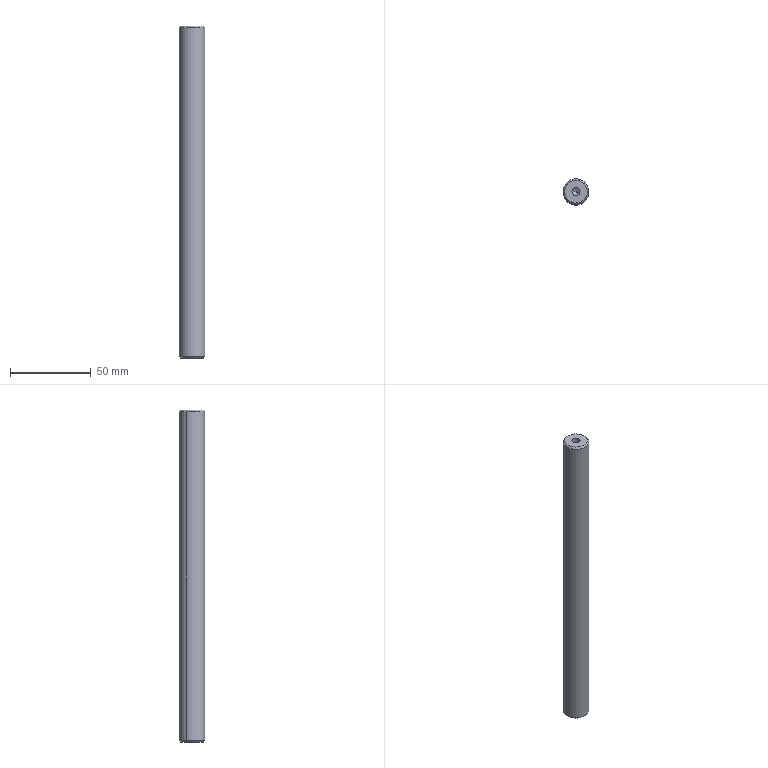Component | SolidWorks | DZ.KX.203-TC1505-30-09-01-05-02-1 | 1 solid | 16 faces | box 16 x 16 x 205 mm | volume 40443 mm3 | cone 8 | cylinder 6 | plane 2 | commonest cylinder face diameters 5 x4 16 x2 | material Malleable Cast Iron
build123d program:
from build123d import *

# Parameters (mm, degrees)
SKETCH1_R             = 8
BOSS_EXTRUDE1_DEPTH   = 205
M6_TAPPED_HOLE1_D     = 5
M6_TAPPED_HOLE1_DEPTH = 18
M6_TAPPED_HOLE1_TIP   = 1.502
M6_TAPPED_HOLE2_D     = 5
M6_TAPPED_HOLE2_DEPTH = 18
M6_TAPPED_HOLE2_TIP   = 1.502
CHAMFER2_SIZE         = 1


with BuildPart() as part:
    # Sketch1 → Boss-Extrude1 (new body)
    with BuildSketch(Plane(origin=(0, 0, 0), x_dir=(0, 0, -1), z_dir=(1, 0, 0))):
        with Locations(Location((0, 0, 0), (0, 0, 180))):
            Circle(SKETCH1_R)
    extrude(amount=BOSS_EXTRUDE1_DEPTH)

    # M6 Tapped Hole1
    with Locations(Plane.ZY):
        with Locations((0, 0)):
            Hole(M6_TAPPED_HOLE1_D / 2, depth=M6_TAPPED_HOLE1_DEPTH)
            with Locations((0, 0, -(M6_TAPPED_HOLE1_DEPTH + M6_TAPPED_HOLE1_TIP / 2))):  # 118° drill point
                Cone(0, M6_TAPPED_HOLE1_D / 2, M6_TAPPED_HOLE1_TIP, mode=Mode.SUBTRACT)

    # M6 Tapped Hole2
    with Locations(Plane(origin=(205, 0, 0), x_dir=(0, 0, -1), z_dir=(1, 0, 0))):
        with Locations((0, 0)):
            Hole(M6_TAPPED_HOLE2_D / 2, depth=M6_TAPPED_HOLE2_DEPTH)
            with Locations((0, 0, -(M6_TAPPED_HOLE2_DEPTH + M6_TAPPED_HOLE2_TIP / 2))):  # 118° drill point
                Cone(0, M6_TAPPED_HOLE2_D / 2, M6_TAPPED_HOLE2_TIP, mode=Mode.SUBTRACT)

    # Chamfer2
    chamfer2_edges = [part.edges().sort_by_distance(p)[0] for p in [
        (0, 0, -8),
        (205, 0, -8),
    ]]
    chamfer(chamfer2_edges, length=CHAMFER2_SIZE)


solid = part.part

# Placed as in the assembly
solid = solid.moved(Location((277, -610.807, 213.06), (0, 90, 0)))
STEP:
#1=COLOUR_RGB('',0.7922,0.8196,0.9333);
#2=FILL_AREA_STYLE_COLOUR('',#1);
#3=FILL_AREA_STYLE('',(#2));
#4=SURFACE_STYLE_FILL_AREA(#3);
#5=SURFACE_SIDE_STYLE('',(#4));
#6=SURFACE_STYLE_USAGE(.BOTH.,#5);
#7=PRESENTATION_STYLE_ASSIGNMENT((#6));
#8=CARTESIAN_POINT('',(11.154,-24.167,0.3173));
#9=VERTEX_POINT('',#8);
#10=CARTESIAN_POINT('',(10.657,-23.928,0.3173));
#11=VERTEX_POINT('',#10);
#12=CARTESIAN_POINT('',(10.906,-24.048,0.3173));
#13=DIRECTION('',(-0.,-0.,-1.));
#14=DIRECTION('',(-0.9007,0.4345,-0.));
#15=AXIS2_PLACEMENT_3D('',#12,#13,#14);
#16=CIRCLE('',#15,0.2756);
#17=EDGE_CURVE('',#9,#11,#16,.T.);
#18=ORIENTED_EDGE('',*,*,#17,.F.);
#19=CARTESIAN_POINT('',(11.189,-24.184,0.3567));
#20=VERTEX_POINT('',#19);
#21=CARTESIAN_POINT('',(11.189,-24.184,0.3567));
#22=DIRECTION('',(0.6369,-0.3073,0.7071));
#23=VECTOR('',#22,39.37);
#24=LINE('',#21,#23);
#25=EDGE_CURVE('',#9,#20,#24,.T.);
#26=ORIENTED_EDGE('',*,*,#25,.T.);
#27=CARTESIAN_POINT('',(10.622,-23.911,0.3567));
#28=VERTEX_POINT('',#27);
#29=CARTESIAN_POINT('',(10.906,-24.048,0.3567));
#30=DIRECTION('',(0.,0.,1.));
#31=DIRECTION('',(-0.9007,0.4345,-0.));
#32=AXIS2_PLACEMENT_3D('',#29,#30,#31);
#33=CIRCLE('',#32,0.315);
#34=EDGE_CURVE('',#28,#20,#33,.T.);
#35=ORIENTED_EDGE('',*,*,#34,.F.);
#36=CARTESIAN_POINT('',(10.622,-23.911,0.3567));
#37=DIRECTION('',(-0.6369,0.3073,0.7071));
#38=VECTOR('',#37,39.37);
#39=LINE('',#36,#38);
#40=EDGE_CURVE('',#11,#28,#39,.T.);
#41=ORIENTED_EDGE('',*,*,#40,.F.);
#42=EDGE_LOOP('',(#18,#26,#35,#41));
#43=FACE_OUTER_BOUND('',#42,.T.);
#44=CARTESIAN_POINT('',(10.906,-24.048,0.3567));
#45=DIRECTION('',(0.,0.,1.));
#46=DIRECTION('',(-0.9007,0.4345,-0.));
#47=AXIS2_PLACEMENT_3D('',#44,#45,#46);
#48=CONICAL_SURFACE('',#47,0.315,0.7854);
#49=ADVANCED_FACE('',(#43),#48,.T.);
#50=CARTESIAN_POINT('',(10.657,-23.928,8.388));
#51=VERTEX_POINT('',#50);
#52=CARTESIAN_POINT('',(11.154,-24.167,8.388));
#53=VERTEX_POINT('',#52);
#54=CARTESIAN_POINT('',(10.906,-24.048,8.388));
#55=DIRECTION('',(0.,0.,1.));
#56=DIRECTION('',(-0.9007,0.4345,0.));
#57=AXIS2_PLACEMENT_3D('',#54,#55,#56);
#58=CIRCLE('',#57,0.2756);
#59=EDGE_CURVE('',#51,#53,#58,.T.);
#60=ORIENTED_EDGE('',*,*,#59,.F.);
#61=CARTESIAN_POINT('',(10.622,-23.911,8.349));
#62=VERTEX_POINT('',#61);
#63=CARTESIAN_POINT('',(10.657,-23.928,8.388));
#64=DIRECTION('',(-0.6369,0.3073,-0.7071));
#65=VECTOR('',#64,39.37);
#66=LINE('',#63,#65);
#67=EDGE_CURVE('',#51,#62,#66,.T.);
#68=ORIENTED_EDGE('',*,*,#67,.T.);
#69=CARTESIAN_POINT('',(11.189,-24.184,8.349));
#70=VERTEX_POINT('',#69);
#71=CARTESIAN_POINT('',(10.906,-24.048,8.349));
#72=DIRECTION('',(-0.,-0.,-1.));
#73=DIRECTION('',(-0.9007,0.4345,0.));
#74=AXIS2_PLACEMENT_3D('',#71,#72,#73);
#75=CIRCLE('',#74,0.315);
#76=EDGE_CURVE('',#70,#62,#75,.T.);
#77=ORIENTED_EDGE('',*,*,#76,.F.);
#78=CARTESIAN_POINT('',(11.154,-24.167,8.388));
#79=DIRECTION('',(0.6369,-0.3073,-0.7071));
#80=VECTOR('',#79,39.37);
#81=LINE('',#78,#80);
#82=EDGE_CURVE('',#53,#70,#81,.T.);
#83=ORIENTED_EDGE('',*,*,#82,.F.);
#84=EDGE_LOOP('',(#60,#68,#77,#83));
#85=FACE_OUTER_BOUND('',#84,.T.);
#86=CARTESIAN_POINT('',(10.906,-24.048,8.388));
#87=DIRECTION('',(-0.,-0.,-1.));
#88=DIRECTION('',(0.9007,-0.4345,0.));
#89=AXIS2_PLACEMENT_3D('',#86,#87,#88);
#90=CONICAL_SURFACE('',#89,0.2756,0.7854);
#91=ADVANCED_FACE('',(#85),#90,.T.);
#92=CARTESIAN_POINT('',(10.994,-24.09,7.68));
#93=VERTEX_POINT('',#92);
#94=CARTESIAN_POINT('',(10.817,-24.005,7.68));
#95=VERTEX_POINT('',#94);
#96=CARTESIAN_POINT('',(10.906,-24.048,7.68));
#97=DIRECTION('',(0.,0.,1.));
#98=DIRECTION('',(-0.9007,0.4345,0.));
#99=AXIS2_PLACEMENT_3D('',#96,#97,#98);
#100=CIRCLE('',#99,0.09843);
#101=EDGE_CURVE('',#93,#95,#100,.T.);
#102=ORIENTED_EDGE('',*,*,#101,.F.);
#103=CARTESIAN_POINT('',(10.994,-24.09,8.388));
#104=VERTEX_POINT('',#103);
#105=CARTESIAN_POINT('',(10.994,-24.09,8.388));
#106=DIRECTION('',(0.,0.,1.));
#107=VECTOR('',#106,39.37);
#108=LINE('',#105,#107);
#109=EDGE_CURVE('',#93,#104,#108,.T.);
#110=ORIENTED_EDGE('',*,*,#109,.T.);
#111=CARTESIAN_POINT('',(10.817,-24.005,8.388));
#112=VERTEX_POINT('',#111);
#113=CARTESIAN_POINT('',(10.906,-24.048,8.388));
#114=DIRECTION('',(0.,0.,1.));
#115=DIRECTION('',(-0.9007,0.4345,0.));
#116=AXIS2_PLACEMENT_3D('',#113,#114,#115);
#117=CIRCLE('',#116,0.09843);
#118=EDGE_CURVE('',#104,#112,#117,.T.);
#119=ORIENTED_EDGE('',*,*,#118,.T.);
#120=CARTESIAN_POINT('',(10.817,-24.005,8.388));
#121=DIRECTION('',(0.,0.,1.));
#122=VECTOR('',#121,39.37);
#123=LINE('',#120,#122);
#124=EDGE_CURVE('',#95,#112,#123,.T.);
#125=ORIENTED_EDGE('',*,*,#124,.F.);
#126=EDGE_LOOP('',(#102,#110,#119,#125));
#127=FACE_OUTER_BOUND('',#126,.T.);
#128=CARTESIAN_POINT('',(10.906,-24.048,8.388));
#129=DIRECTION('',(0.,0.,1.));
#130=DIRECTION('',(-0.9007,0.4345,0.));
#131=AXIS2_PLACEMENT_3D('',#128,#129,#130);
#132=CYLINDRICAL_SURFACE('',#131,0.09843);
#133=ADVANCED_FACE('',(#127),#132,.F.);
#134=CARTESIAN_POINT('',(10.906,-24.048,7.62));
#135=VERTEX_POINT('',#134);
#136=CARTESIAN_POINT('',(10.817,-24.005,7.68));
#137=DIRECTION('',(-0.772,0.3725,0.515));
#138=VECTOR('',#137,39.37);
#139=LINE('',#136,#138);
#140=EDGE_CURVE('',#135,#95,#139,.T.);
#141=ORIENTED_EDGE('',*,*,#140,.F.);
#142=CARTESIAN_POINT('',(10.994,-24.09,7.68));
#143=DIRECTION('',(0.772,-0.3725,0.515));
#144=VECTOR('',#143,39.37);
#145=LINE('',#142,#144);
#146=EDGE_CURVE('',#135,#93,#145,.T.);
#147=ORIENTED_EDGE('',*,*,#146,.T.);
#148=ORIENTED_EDGE('',*,*,#101,.T.);
#149=EDGE_LOOP('',(#141,#147,#148));
#150=FACE_OUTER_BOUND('',#149,.T.);
#151=CARTESIAN_POINT('',(10.906,-24.048,7.68));
#152=DIRECTION('',(0.,0.,1.));
#153=DIRECTION('',(-0.9007,0.4345,0.));
#154=AXIS2_PLACEMENT_3D('',#151,#152,#153);
#155=CONICAL_SURFACE('',#154,0.09843,1.03);
#156=ADVANCED_FACE('',(#150),#155,.F.);
#157=CARTESIAN_POINT('',(10.817,-24.005,1.026));
#158=VERTEX_POINT('',#157);
#159=CARTESIAN_POINT('',(10.994,-24.09,1.026));
#160=VERTEX_POINT('',#159);
#161=CARTESIAN_POINT('',(10.906,-24.048,1.026));
#162=DIRECTION('',(-0.,-0.,-1.));
#163=DIRECTION('',(0.9007,-0.4345,0.));
#164=AXIS2_PLACEMENT_3D('',#161,#162,#163);
#165=CIRCLE('',#164,0.09843);
#166=EDGE_CURVE('',#158,#160,#165,.T.);
#167=ORIENTED_EDGE('',*,*,#166,.F.);
#168=CARTESIAN_POINT('',(10.817,-24.005,0.3173));
#169=VERTEX_POINT('',#168);
#170=CARTESIAN_POINT('',(10.817,-24.005,0.3173));
#171=DIRECTION('',(-0.,-0.,-1.));
#172=VECTOR('',#171,39.37);
#173=LINE('',#170,#172);
#174=EDGE_CURVE('',#158,#169,#173,.T.);
#175=ORIENTED_EDGE('',*,*,#174,.T.);
#176=CARTESIAN_POINT('',(10.994,-24.09,0.3173));
#177=VERTEX_POINT('',#176);
#178=CARTESIAN_POINT('',(10.906,-24.048,0.3173));
#179=DIRECTION('',(-0.,-0.,-1.));
#180=DIRECTION('',(0.9007,-0.4345,0.));
#181=AXIS2_PLACEMENT_3D('',#178,#179,#180);
#182=CIRCLE('',#181,0.09843);
#183=EDGE_CURVE('',#169,#177,#182,.T.);
#184=ORIENTED_EDGE('',*,*,#183,.T.);
#185=CARTESIAN_POINT('',(10.994,-24.09,0.3173));
#186=DIRECTION('',(-0.,-0.,-1.));
#187=VECTOR('',#186,39.37);
#188=LINE('',#185,#187);
#189=EDGE_CURVE('',#160,#177,#188,.T.);
#190=ORIENTED_EDGE('',*,*,#189,.F.);
#191=EDGE_LOOP('',(#167,#175,#184,#190));
#192=FACE_OUTER_BOUND('',#191,.T.);
#193=CARTESIAN_POINT('',(10.906,-24.048,0.3173));
#194=DIRECTION('',(-0.,-0.,-1.));
#195=DIRECTION('',(0.9007,-0.4345,0.));
#196=AXIS2_PLACEMENT_3D('',#193,#194,#195);
#197=CYLINDRICAL_SURFACE('',#196,0.09843);
#198=ADVANCED_FACE('',(#192),#197,.F.);
#199=CARTESIAN_POINT('',(10.906,-24.048,1.085));
#200=VERTEX_POINT('',#199);
#201=CARTESIAN_POINT('',(10.994,-24.09,1.026));
#202=DIRECTION('',(0.772,-0.3725,-0.515));
#203=VECTOR('',#202,39.37);
#204=LINE('',#201,#203);
#205=EDGE_CURVE('',#200,#160,#204,.T.);
#206=ORIENTED_EDGE('',*,*,#205,.F.);
#207=CARTESIAN_POINT('',(10.817,-24.005,1.026));
#208=DIRECTION('',(-0.772,0.3725,-0.515));
#209=VECTOR('',#208,39.37);
#210=LINE('',#207,#209);
#211=EDGE_CURVE('',#200,#158,#210,.T.);
#212=ORIENTED_EDGE('',*,*,#211,.T.);
#213=ORIENTED_EDGE('',*,*,#166,.T.);
#214=EDGE_LOOP('',(#206,#212,#213));
#215=FACE_OUTER_BOUND('',#214,.T.);
#216=CARTESIAN_POINT('',(10.906,-24.048,1.026));
#217=DIRECTION('',(-0.,-0.,-1.));
#218=DIRECTION('',(0.9007,-0.4345,0.));
#219=AXIS2_PLACEMENT_3D('',#216,#217,#218);
#220=CONICAL_SURFACE('',#219,0.09843,1.03);
#221=ADVANCED_FACE('',(#215),#220,.F.);
#222=ORIENTED_EDGE('',*,*,#76,.T.);
#223=CARTESIAN_POINT('',(10.622,-23.911,8.388));
#224=DIRECTION('',(-0.,-0.,-1.));
#225=VECTOR('',#224,39.37);
#226=LINE('',#223,#225);
#227=EDGE_CURVE('',#62,#28,#226,.T.);
#228=ORIENTED_EDGE('',*,*,#227,.T.);
#229=ORIENTED_EDGE('',*,*,#34,.T.);
#230=CARTESIAN_POINT('',(11.189,-24.184,8.388));
#231=DIRECTION('',(-0.,-0.,-1.));
#232=VECTOR('',#231,39.37);
#233=LINE('',#230,#232);
#234=EDGE_CURVE('',#70,#20,#233,.T.);
#235=ORIENTED_EDGE('',*,*,#234,.F.);
#236=EDGE_LOOP('',(#222,#228,#229,#235));
#237=FACE_OUTER_BOUND('',#236,.T.);
#238=CARTESIAN_POINT('',(10.906,-24.048,8.388));
#239=DIRECTION('',(-0.,-0.,-1.));
#240=DIRECTION('',(0.9007,-0.4345,0.));
#241=AXIS2_PLACEMENT_3D('',#238,#239,#240);
#242=CYLINDRICAL_SURFACE('',#241,0.315);
#243=ADVANCED_FACE('',(#237),#242,.T.);
#244=ORIENTED_EDGE('',*,*,#227,.F.);
#245=CARTESIAN_POINT('',(10.906,-24.048,8.349));
#246=DIRECTION('',(-0.,-0.,-1.));
#247=DIRECTION('',(-0.9007,0.4345,0.));
#248=AXIS2_PLACEMENT_3D('',#245,#246,#247);
#249=CIRCLE('',#248,0.315);
#250=EDGE_CURVE('',#62,#70,#249,.T.);
#251=ORIENTED_EDGE('',*,*,#250,.T.);
#252=ORIENTED_EDGE('',*,*,#234,.T.);
#253=CARTESIAN_POINT('',(10.906,-24.048,0.3567));
#254=DIRECTION('',(0.,0.,1.));
#255=DIRECTION('',(-0.9007,0.4345,-0.));
#256=AXIS2_PLACEMENT_3D('',#253,#254,#255);
#257=CIRCLE('',#256,0.315);
#258=EDGE_CURVE('',#20,#28,#257,.T.);
#259=ORIENTED_EDGE('',*,*,#258,.T.);
#260=EDGE_LOOP('',(#244,#251,#252,#259));
#261=FACE_OUTER_BOUND('',#260,.T.);
#262=CARTESIAN_POINT('',(10.906,-24.048,8.388));
#263=DIRECTION('',(-0.,-0.,-1.));
#264=DIRECTION('',(0.9007,-0.4345,0.));
#265=AXIS2_PLACEMENT_3D('',#262,#263,#264);
#266=CYLINDRICAL_SURFACE('',#265,0.315);
#267=ADVANCED_FACE('',(#261),#266,.T.);
#268=CARTESIAN_POINT('',(10.906,-24.048,8.388));
#269=DIRECTION('',(0.,0.,1.));
#270=DIRECTION('',(-0.9007,0.4345,0.));
#271=AXIS2_PLACEMENT_3D('',#268,#269,#270);
#272=CIRCLE('',#271,0.2756);
#273=EDGE_CURVE('',#53,#51,#272,.T.);
#274=ORIENTED_EDGE('',*,*,#273,.T.);
#275=ORIENTED_EDGE('',*,*,#59,.T.);
#276=EDGE_LOOP('',(#274,#275));
#277=FACE_OUTER_BOUND('',#276,.T.);
#278=CARTESIAN_POINT('',(10.906,-24.048,8.388));
#279=DIRECTION('',(0.,0.,1.));
#280=DIRECTION('',(-0.9007,0.4345,0.));
#281=AXIS2_PLACEMENT_3D('',#278,#279,#280);
#282=CIRCLE('',#281,0.09843);
#283=EDGE_CURVE('',#112,#104,#282,.T.);
#284=ORIENTED_EDGE('',*,*,#283,.F.);
#285=ORIENTED_EDGE('',*,*,#118,.F.);
#286=EDGE_LOOP('',(#284,#285));
#287=FACE_BOUND('',#286,.T.);
#288=CARTESIAN_POINT('',(10.906,-24.048,8.388));
#289=DIRECTION('',(0.,0.,1.));
#290=DIRECTION('',(-0.9007,0.4345,-0.));
#291=AXIS2_PLACEMENT_3D('',#288,#289,#290);
#292=PLANE('',#291);
#293=ADVANCED_FACE('',(#277,#287),#292,.T.);
#294=CARTESIAN_POINT('',(10.906,-24.048,0.3173));
#295=DIRECTION('',(-0.,-0.,-1.));
#296=DIRECTION('',(-0.9007,0.4345,-0.));
#297=AXIS2_PLACEMENT_3D('',#294,#295,#296);
#298=CIRCLE('',#297,0.2756);
#299=EDGE_CURVE('',#11,#9,#298,.T.);
#300=ORIENTED_EDGE('',*,*,#299,.T.);
#301=ORIENTED_EDGE('',*,*,#17,.T.);
#302=EDGE_LOOP('',(#300,#301));
#303=FACE_OUTER_BOUND('',#302,.T.);
#304=CARTESIAN_POINT('',(10.906,-24.048,0.3173));
#305=DIRECTION('',(-0.,-0.,-1.));
#306=DIRECTION('',(0.9007,-0.4345,0.));
#307=AXIS2_PLACEMENT_3D('',#304,#305,#306);
#308=CIRCLE('',#307,0.09843);
#309=EDGE_CURVE('',#177,#169,#308,.T.);
#310=ORIENTED_EDGE('',*,*,#309,.F.);
#311=ORIENTED_EDGE('',*,*,#183,.F.);
#312=EDGE_LOOP('',(#310,#311));
#313=FACE_BOUND('',#312,.T.);
#314=CARTESIAN_POINT('',(10.906,-24.048,0.3173));
#315=DIRECTION('',(0.,0.,1.));
#316=DIRECTION('',(-0.9007,0.4345,-0.));
#317=AXIS2_PLACEMENT_3D('',#314,#315,#316);
#318=PLANE('',#317);
#319=ADVANCED_FACE('',(#303,#313),#318,.F.);
#320=ORIENTED_EDGE('',*,*,#211,.F.);
#321=ORIENTED_EDGE('',*,*,#205,.T.);
#322=CARTESIAN_POINT('',(10.906,-24.048,1.026));
#323=DIRECTION('',(-0.,-0.,-1.));
#324=DIRECTION('',(0.9007,-0.4345,0.));
#325=AXIS2_PLACEMENT_3D('',#322,#323,#324);
#326=CIRCLE('',#325,0.09843);
#327=EDGE_CURVE('',#160,#158,#326,.T.);
#328=ORIENTED_EDGE('',*,*,#327,.T.);
#329=EDGE_LOOP('',(#320,#321,#328));
#330=FACE_OUTER_BOUND('',#329,.T.);
#331=CARTESIAN_POINT('',(10.906,-24.048,1.026));
#332=DIRECTION('',(-0.,-0.,-1.));
#333=DIRECTION('',(0.9007,-0.4345,0.));
#334=AXIS2_PLACEMENT_3D('',#331,#332,#333);
#335=CONICAL_SURFACE('',#334,0.09843,1.03);
#336=ADVANCED_FACE('',(#330),#335,.F.);
#337=ORIENTED_EDGE('',*,*,#174,.F.);
#338=ORIENTED_EDGE('',*,*,#327,.F.);
#339=ORIENTED_EDGE('',*,*,#189,.T.);
#340=ORIENTED_EDGE('',*,*,#309,.T.);
#341=EDGE_LOOP('',(#337,#338,#339,#340));
#342=FACE_OUTER_BOUND('',#341,.T.);
#343=CARTESIAN_POINT('',(10.906,-24.048,0.3173));
#344=DIRECTION('',(-0.,-0.,-1.));
#345=DIRECTION('',(0.9007,-0.4345,0.));
#346=AXIS2_PLACEMENT_3D('',#343,#344,#345);
#347=CYLINDRICAL_SURFACE('',#346,0.09843);
#348=ADVANCED_FACE('',(#342),#347,.F.);
#349=ORIENTED_EDGE('',*,*,#146,.F.);
#350=ORIENTED_EDGE('',*,*,#140,.T.);
#351=CARTESIAN_POINT('',(10.906,-24.048,7.68));
#352=DIRECTION('',(0.,0.,1.));
#353=DIRECTION('',(-0.9007,0.4345,0.));
#354=AXIS2_PLACEMENT_3D('',#351,#352,#353);
#355=CIRCLE('',#354,0.09843);
#356=EDGE_CURVE('',#95,#93,#355,.T.);
#357=ORIENTED_EDGE('',*,*,#356,.T.);
#358=EDGE_LOOP('',(#349,#350,#357));
#359=FACE_OUTER_BOUND('',#358,.T.);
#360=CARTESIAN_POINT('',(10.906,-24.048,7.68));
#361=DIRECTION('',(0.,0.,1.));
#362=DIRECTION('',(-0.9007,0.4345,0.));
#363=AXIS2_PLACEMENT_3D('',#360,#361,#362);
#364=CONICAL_SURFACE('',#363,0.09843,1.03);
#365=ADVANCED_FACE('',(#359),#364,.F.);
#366=ORIENTED_EDGE('',*,*,#109,.F.);
#367=ORIENTED_EDGE('',*,*,#356,.F.);
#368=ORIENTED_EDGE('',*,*,#124,.T.);
#369=ORIENTED_EDGE('',*,*,#283,.T.);
#370=EDGE_LOOP('',(#366,#367,#368,#369));
#371=FACE_OUTER_BOUND('',#370,.T.);
#372=CARTESIAN_POINT('',(10.906,-24.048,8.388));
#373=DIRECTION('',(0.,0.,1.));
#374=DIRECTION('',(-0.9007,0.4345,0.));
#375=AXIS2_PLACEMENT_3D('',#372,#373,#374);
#376=CYLINDRICAL_SURFACE('',#375,0.09843);
#377=ADVANCED_FACE('',(#371),#376,.F.);
#378=ORIENTED_EDGE('',*,*,#67,.F.);
#379=ORIENTED_EDGE('',*,*,#273,.F.);
#380=ORIENTED_EDGE('',*,*,#82,.T.);
#381=ORIENTED_EDGE('',*,*,#250,.F.);
#382=EDGE_LOOP('',(#378,#379,#380,#381));
#383=FACE_OUTER_BOUND('',#382,.T.);
#384=CARTESIAN_POINT('',(10.906,-24.048,8.388));
#385=DIRECTION('',(-0.,-0.,-1.));
#386=DIRECTION('',(0.9007,-0.4345,0.));
#387=AXIS2_PLACEMENT_3D('',#384,#385,#386);
#388=CONICAL_SURFACE('',#387,0.2756,0.7854);
#389=ADVANCED_FACE('',(#383),#388,.T.);
#390=ORIENTED_EDGE('',*,*,#25,.F.);
#391=ORIENTED_EDGE('',*,*,#299,.F.);
#392=ORIENTED_EDGE('',*,*,#40,.T.);
#393=ORIENTED_EDGE('',*,*,#258,.F.);
#394=EDGE_LOOP('',(#390,#391,#392,#393));
#395=FACE_OUTER_BOUND('',#394,.T.);
#396=CARTESIAN_POINT('',(10.906,-24.048,0.3567));
#397=DIRECTION('',(0.,0.,1.));
#398=DIRECTION('',(-0.9007,0.4345,-0.));
#399=AXIS2_PLACEMENT_3D('',#396,#397,#398);
#400=CONICAL_SURFACE('',#399,0.315,0.7854);
#401=ADVANCED_FACE('',(#395),#400,.T.);
#402=CLOSED_SHELL('',(#49,#91,#133,#156,#198,#221,#243,#267,#293,#319,#336,#348,#365,#377,#389,#401));
#403=MANIFOLD_SOLID_BREP('',#402);
#404=STYLED_ITEM('',(#7),#403);
#405=PRESENTATION_LAYER_ASSIGNMENT('','',(#404));
#406=CARTESIAN_POINT('',(0.,0.,0.));
#407=DIRECTION('',(0.,0.,1.));
#408=DIRECTION('',(1.,0.,0.));
#409=AXIS2_PLACEMENT_3D('',#406,#407,#408);
#410=(LENGTH_UNIT()NAMED_UNIT(*)SI_UNIT($,.METRE.));
#411=LENGTH_MEASURE_WITH_UNIT(LENGTH_MEASURE(0.0254),#410);
#412=DIMENSIONAL_EXPONENTS(1.,0.,0.,0.,0.,0.,0.);
#413=(CONVERSION_BASED_UNIT('',#411)LENGTH_UNIT()NAMED_UNIT(#412));
#414=UNCERTAINTY_MEASURE_WITH_UNIT(LENGTH_MEASURE(0.00001),#413,'','');
#415=(NAMED_UNIT(*)PLANE_ANGLE_UNIT()SI_UNIT($,.RADIAN.));
#416=(NAMED_UNIT(*)SI_UNIT($,.STERADIAN.)SOLID_ANGLE_UNIT());
#417=(GEOMETRIC_REPRESENTATION_CONTEXT(3)GLOBAL_UNCERTAINTY_ASSIGNED_CONTEXT((#414))GLOBAL_UNIT_ASSIGNED_CONTEXT((#413,#415,#416))REPRESENTATION_CONTEXT('',''));
#418=ADVANCED_BREP_SHAPE_REPRESENTATION('',(#403,#409),#417);
#419=(LENGTH_UNIT()NAMED_UNIT(*)SI_UNIT($,.METRE.));
#420=LENGTH_MEASURE_WITH_UNIT(LENGTH_MEASURE(0.0254),#419);
#421=DIMENSIONAL_EXPONENTS(1.,0.,0.,0.,0.,0.,0.);
#422=(CONVERSION_BASED_UNIT('',#420)LENGTH_UNIT()NAMED_UNIT(#421));
#423=UNCERTAINTY_MEASURE_WITH_UNIT(LENGTH_MEASURE(0.00001),#422,'','');
#424=(NAMED_UNIT(*)PLANE_ANGLE_UNIT()SI_UNIT($,.RADIAN.));
#425=(NAMED_UNIT(*)SI_UNIT($,.STERADIAN.)SOLID_ANGLE_UNIT());
#426=(GEOMETRIC_REPRESENTATION_CONTEXT(3)GLOBAL_UNCERTAINTY_ASSIGNED_CONTEXT((#423))GLOBAL_UNIT_ASSIGNED_CONTEXT((#422,#424,#425))REPRESENTATION_CONTEXT('',''));
#427=MECHANICAL_DESIGN_GEOMETRIC_PRESENTATION_REPRESENTATION('',(#404),#426);